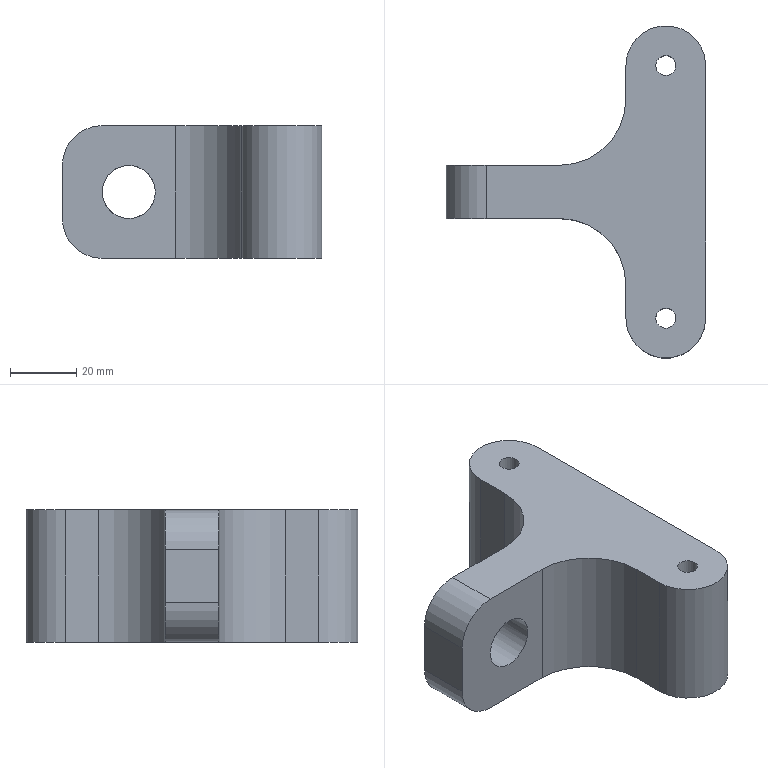Component | NX | FRONT_BRACKET | 1 solid | 17 faces | volume 126047 mm3 | cylinder 9 | plane 8 | commonest cylinder face diameters 24 x4 40 x2 6 x2 16 x1